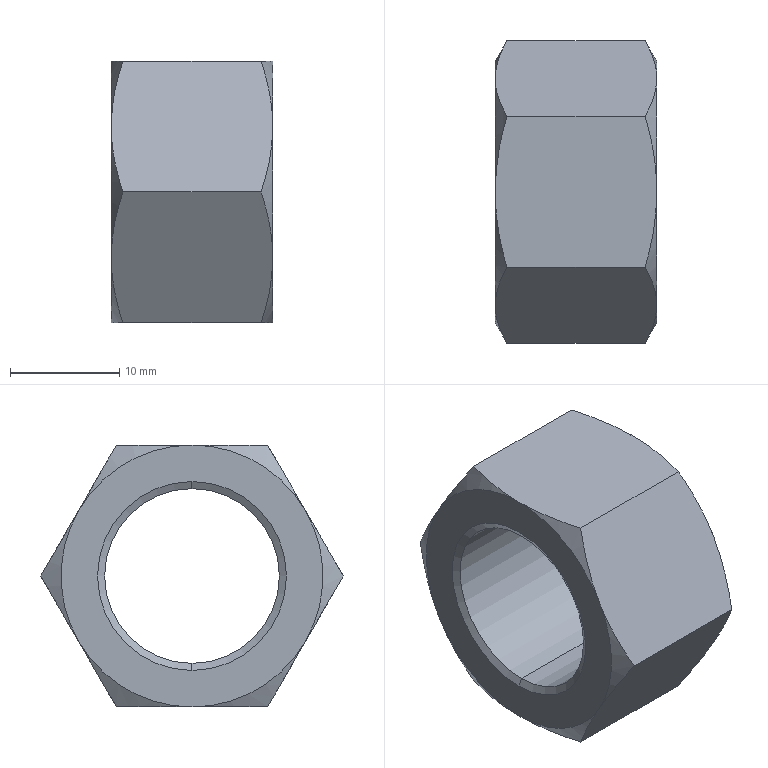Component | SolidWorks | GB_T6170-2015[Type1HexNutM16]-1 | 1 solid | 26 faces | box 14.8 x 27.71 x 24 mm | volume 4364 mm3 | cone 16 | plane 8 | cylinder 2 | commonest cylinder face diameters 16 x2
build123d program:
from build123d import *

# Parameters (mm, degrees)
SKETCH3_R               = 6.918
BOSS_EXTRUDE1_DEPTH     = 14.8
SKETCH5_R               = 20.062
SKETCH5_R_2             = 12
CUT_EXTRUDE1_2_DEPTH    = 2.96
CUT_EXTRUDE1_2_DRAFT    = -60
SKETCH7_R               = 20.062
SKETCH7_R_2             = 12
CUT_EXTRUDE2_DEPTH      = 2.96
CUT_EXTRUDE2_DRAFT      = -60
CUT_EXTRUDE1_DEPTH      = 24.559
CUT_EXTRUDE1_DEPTH_BACK = 24.559
SKETCH1_R               = 8


with BuildPart() as part:
    # Sketch3 → Boss-Extrude1 (new body)
    with BuildSketch(Plane.XY):
        Polygon((0, 13.856), (-12, 6.928), (-12, -6.928), (0, -13.856), (12, -6.928), (12, 6.928), align=None)
        Circle(SKETCH3_R, mode=Mode.SUBTRACT)
    extrude(amount=-BOSS_EXTRUDE1_DEPTH)

    # Sketch4 → Cut-Revolve1 (revolve, cut)
    with BuildSketch(Plane(origin=(0, 0, 0), x_dir=(0, 0, -1), z_dir=(1, 0, 0)), mode=Mode.PRIVATE) as cut_revolve1_sk:
        Polygon((0, 8.65), (1, 6.918), (1, 0), (0, 0), align=None)
        Polygon((14.8, 0), (14.8, 8.65), (13.8, 6.918), (13.8, 0), align=None)
    revolve(cut_revolve1_sk.sketch.rotate(Axis((0, 0, 0), (0, 0, -1)), 90), axis=Axis((0, 0, 0), (0, 0, -1)), mode=Mode.SUBTRACT)


with BuildPart() as cut_extrude1_2_tool:
    # Sketch5 → Cut-Extrude1_2 (with draft: the straight prism first)
    with BuildSketch(Plane.XY):
        Circle(SKETCH5_R)
        Circle(SKETCH5_R_2, mode=Mode.SUBTRACT)
    extrude(amount=-CUT_EXTRUDE1_2_DEPTH)
    # Cut-Extrude1_2: the draft: its side faces are tilted about the plane it starts from
    cut_extrude1_2_sides = [cut_extrude1_2_tool.faces().sort_by_distance(p)[0] for p in [
        (-20.062, 0, -1.48),
        (-12, 0, -1.48),
    ]]
    draft(cut_extrude1_2_sides, Plane.XY, CUT_EXTRUDE1_2_DRAFT)


with BuildPart() as part_1:
    add(part.part)

    # Cut-Extrude1_2: cut by cut_extrude1_2_tool
    add(cut_extrude1_2_tool.part, mode=Mode.SUBTRACT)


with BuildPart() as cut_extrude2_tool:
    # Sketch7 → Cut-Extrude2 (with draft: the straight prism first)
    with BuildSketch(Plane(origin=(0, 0, -14.8), x_dir=(-1, 0, 0), z_dir=(0, 0, -1))):
        Circle(SKETCH7_R)
        Circle(SKETCH7_R_2, mode=Mode.SUBTRACT)
    extrude(amount=-CUT_EXTRUDE2_DEPTH)
    # Cut-Extrude2: the draft: its side faces are tilted about the plane it starts from
    cut_extrude2_sides = [cut_extrude2_tool.faces().sort_by_distance(p)[0] for p in [
        (20.062, 0, -13.32),
        (12, 0, -13.32),
    ]]
    draft(cut_extrude2_sides, Plane(origin=(0, 0, -14.8), x_dir=(-1, 0, 0), z_dir=(0, 0, -1)), CUT_EXTRUDE2_DRAFT)


with BuildPart() as part_2:
    add(part_1.part)

    # Cut-Extrude2: cut by cut_extrude2_tool
    add(cut_extrude2_tool.part, mode=Mode.SUBTRACT)

    # Sketch1 → Cut-Extrude1 (cut, two sides: drawn at the far end of the back side and taken through both)
    with BuildSketch(Plane.XY.offset(-CUT_EXTRUDE1_DEPTH_BACK)):
        Circle(SKETCH1_R)
    extrude(amount=CUT_EXTRUDE1_DEPTH + CUT_EXTRUDE1_DEPTH_BACK, mode=Mode.SUBTRACT)


solid = part_2.part

# Placed as in the assembly
solid = solid.moved(Location((-236.5, 7106.066, 106.066), (0, 90, 0)))
STEP:
#1=COLOUR_RGB('',0.7922,0.8196,0.9333);
#2=FILL_AREA_STYLE_COLOUR('',#1);
#3=FILL_AREA_STYLE('',(#2));
#4=SURFACE_STYLE_FILL_AREA(#3);
#5=SURFACE_SIDE_STYLE('',(#4));
#6=SURFACE_STYLE_USAGE(.BOTH.,#5);
#7=PRESENTATION_STYLE_ASSIGNMENT((#6));
#8=CARTESIAN_POINT('',(-9.326,279.766,4.491));
#9=VERTEX_POINT('',#8);
#10=CARTESIAN_POINT('',(-9.326,279.766,3.861));
#11=VERTEX_POINT('',#10);
#12=CARTESIAN_POINT('',(-9.326,279.766,4.176));
#13=DIRECTION('',(1.,0.,0.));
#14=DIRECTION('',(0.,0.,-1.));
#15=AXIS2_PLACEMENT_3D('',#12,#13,#14);
#16=CIRCLE('',#15,0.315);
#17=EDGE_CURVE('',#9,#11,#16,.T.);
#18=ORIENTED_EDGE('',*,*,#17,.T.);
#19=CARTESIAN_POINT('',(-9.879,279.766,3.861));
#20=VERTEX_POINT('',#19);
#21=CARTESIAN_POINT('',(-9.311,279.766,3.861));
#22=DIRECTION('',(-1.,0.,0.));
#23=VECTOR('',#22,39.37);
#24=LINE('',#21,#23);
#25=EDGE_CURVE('',#11,#20,#24,.T.);
#26=ORIENTED_EDGE('',*,*,#25,.T.);
#27=CARTESIAN_POINT('',(-9.879,279.766,4.491));
#28=VERTEX_POINT('',#27);
#29=CARTESIAN_POINT('',(-9.879,279.766,4.176));
#30=DIRECTION('',(-1.,0.,0.));
#31=DIRECTION('',(0.,0.,1.));
#32=AXIS2_PLACEMENT_3D('',#29,#30,#31);
#33=CIRCLE('',#32,0.315);
#34=EDGE_CURVE('',#20,#28,#33,.T.);
#35=ORIENTED_EDGE('',*,*,#34,.T.);
#36=CARTESIAN_POINT('',(-9.311,279.766,4.491));
#37=DIRECTION('',(-1.,0.,0.));
#38=VECTOR('',#37,39.37);
#39=LINE('',#36,#38);
#40=EDGE_CURVE('',#9,#28,#39,.T.);
#41=ORIENTED_EDGE('',*,*,#40,.F.);
#42=EDGE_LOOP('',(#18,#26,#35,#41));
#43=FACE_OUTER_BOUND('',#42,.T.);
#44=CARTESIAN_POINT('',(-9.311,279.766,4.176));
#45=DIRECTION('',(-1.,0.,0.));
#46=DIRECTION('',(0.,0.,1.));
#47=AXIS2_PLACEMENT_3D('',#44,#45,#46);
#48=CYLINDRICAL_SURFACE('',#47,0.315);
#49=ADVANCED_FACE('',(#43),#48,.F.);
#50=ORIENTED_EDGE('',*,*,#17,.F.);
#51=CARTESIAN_POINT('',(-9.311,279.766,4.516));
#52=VERTEX_POINT('',#51);
#53=CARTESIAN_POINT('',(-9.311,279.766,4.516));
#54=DIRECTION('',(0.5,0.,0.866));
#55=VECTOR('',#54,39.37);
#56=LINE('',#53,#55);
#57=EDGE_CURVE('',#9,#52,#56,.T.);
#58=ORIENTED_EDGE('',*,*,#57,.T.);
#59=CARTESIAN_POINT('',(-9.311,279.766,3.835));
#60=VERTEX_POINT('',#59);
#61=CARTESIAN_POINT('',(-9.311,279.766,4.176));
#62=DIRECTION('',(-1.,0.,0.));
#63=DIRECTION('',(0.,0.,1.));
#64=AXIS2_PLACEMENT_3D('',#61,#62,#63);
#65=CIRCLE('',#64,0.3406);
#66=EDGE_CURVE('',#60,#52,#65,.T.);
#67=ORIENTED_EDGE('',*,*,#66,.F.);
#68=CARTESIAN_POINT('',(-9.311,279.766,3.835));
#69=DIRECTION('',(0.5,0.,-0.866));
#70=VECTOR('',#69,39.37);
#71=LINE('',#68,#70);
#72=EDGE_CURVE('',#11,#60,#71,.T.);
#73=ORIENTED_EDGE('',*,*,#72,.F.);
#74=EDGE_LOOP('',(#50,#58,#67,#73));
#75=FACE_OUTER_BOUND('',#74,.T.);
#76=CARTESIAN_POINT('',(-9.311,279.766,4.176));
#77=DIRECTION('',(1.,0.,0.));
#78=DIRECTION('',(0.,0.,-1.));
#79=AXIS2_PLACEMENT_3D('',#76,#77,#78);
#80=CONICAL_SURFACE('',#79,0.3406,1.047);
#81=ADVANCED_FACE('',(#75),#80,.F.);
#82=ORIENTED_EDGE('',*,*,#34,.F.);
#83=CARTESIAN_POINT('',(-9.894,279.766,3.835));
#84=VERTEX_POINT('',#83);
#85=CARTESIAN_POINT('',(-9.854,279.766,3.903));
#86=DIRECTION('',(-0.5,0.,-0.866));
#87=VECTOR('',#86,39.37);
#88=LINE('',#85,#87);
#89=EDGE_CURVE('',#20,#84,#88,.T.);
#90=ORIENTED_EDGE('',*,*,#89,.T.);
#91=CARTESIAN_POINT('',(-9.894,279.766,4.516));
#92=VERTEX_POINT('',#91);
#93=CARTESIAN_POINT('',(-9.894,279.766,4.176));
#94=DIRECTION('',(-1.,0.,0.));
#95=DIRECTION('',(0.,0.,1.));
#96=AXIS2_PLACEMENT_3D('',#93,#94,#95);
#97=CIRCLE('',#96,0.3406);
#98=EDGE_CURVE('',#84,#92,#97,.T.);
#99=ORIENTED_EDGE('',*,*,#98,.T.);
#100=CARTESIAN_POINT('',(-9.854,279.766,4.448));
#101=DIRECTION('',(-0.5,0.,0.866));
#102=VECTOR('',#101,39.37);
#103=LINE('',#100,#102);
#104=EDGE_CURVE('',#28,#92,#103,.T.);
#105=ORIENTED_EDGE('',*,*,#104,.F.);
#106=EDGE_LOOP('',(#82,#90,#99,#105));
#107=FACE_OUTER_BOUND('',#106,.T.);
#108=CARTESIAN_POINT('',(-9.854,279.766,4.176));
#109=DIRECTION('',(-1.,0.,0.));
#110=DIRECTION('',(0.,0.,1.));
#111=AXIS2_PLACEMENT_3D('',#108,#109,#110);
#112=CONICAL_SURFACE('',#111,0.2723,1.047);
#113=ADVANCED_FACE('',(#107),#112,.F.);
#114=CARTESIAN_POINT('',(-9.353,280.039,4.648));
#115=VERTEX_POINT('',#114);
#116=CARTESIAN_POINT('',(-9.852,280.039,4.648));
#117=VERTEX_POINT('',#116);
#118=CARTESIAN_POINT('',(-9.311,280.039,4.648));
#119=DIRECTION('',(-1.,0.,0.));
#120=VECTOR('',#119,39.37);
#121=LINE('',#118,#120);
#122=EDGE_CURVE('',#115,#117,#121,.T.);
#123=ORIENTED_EDGE('',*,*,#122,.F.);
#124=CARTESIAN_POINT('',(-9.311,280.176,4.412));
#125=VERTEX_POINT('',#124);
#126=CARTESIAN_POINT('',(-9.353,280.039,4.648));
#127=CARTESIAN_POINT('',(-9.34,280.061,4.61));
#128=CARTESIAN_POINT('',(-9.33,280.084,4.571));
#129=CARTESIAN_POINT('',(-9.315,280.129,4.492));
#130=CARTESIAN_POINT('',(-9.311,280.152,4.452));
#131=CARTESIAN_POINT('',(-9.311,280.176,4.412));
#132=B_SPLINE_CURVE_WITH_KNOTS('',3,(#126,#127,#128,#129,#130,#131),.UNSPECIFIED.,.F.,.F.,(4,2,4),(0.00000024,0.003505,0.00701),.UNSPECIFIED.);
#133=EDGE_CURVE('',#115,#125,#132,.T.);
#134=ORIENTED_EDGE('',*,*,#133,.T.);
#135=CARTESIAN_POINT('',(-9.353,280.312,4.176));
#136=VERTEX_POINT('',#135);
#137=CARTESIAN_POINT('',(-9.311,280.176,4.412));
#138=CARTESIAN_POINT('',(-9.311,280.187,4.392));
#139=CARTESIAN_POINT('',(-9.312,280.199,4.372));
#140=CARTESIAN_POINT('',(-9.316,280.222,4.332));
#141=CARTESIAN_POINT('',(-9.319,280.233,4.312));
#142=CARTESIAN_POINT('',(-9.33,280.267,4.253));
#143=CARTESIAN_POINT('',(-9.34,280.29,4.214));
#144=CARTESIAN_POINT('',(-9.353,280.312,4.176));
#145=B_SPLINE_CURVE_WITH_KNOTS('',3,(#137,#138,#139,#140,#141,#142,#143,#144),.UNSPECIFIED.,.F.,.F.,(4,2,2,4),(0.00701,0.008756,0.0105,0.01399),.UNSPECIFIED.);
#146=EDGE_CURVE('',#125,#136,#145,.T.);
#147=ORIENTED_EDGE('',*,*,#146,.T.);
#148=CARTESIAN_POINT('',(-9.852,280.312,4.176));
#149=VERTEX_POINT('',#148);
#150=CARTESIAN_POINT('',(-9.311,280.312,4.176));
#151=DIRECTION('',(-1.,0.,0.));
#152=VECTOR('',#151,39.37);
#153=LINE('',#150,#152);
#154=EDGE_CURVE('',#136,#149,#153,.T.);
#155=ORIENTED_EDGE('',*,*,#154,.T.);
#156=CARTESIAN_POINT('',(-9.894,280.176,4.412));
#157=VERTEX_POINT('',#156);
#158=CARTESIAN_POINT('',(-9.852,280.312,4.176));
#159=CARTESIAN_POINT('',(-9.864,280.29,4.214));
#160=CARTESIAN_POINT('',(-9.875,280.267,4.253));
#161=CARTESIAN_POINT('',(-9.89,280.222,4.332));
#162=CARTESIAN_POINT('',(-9.894,280.199,4.372));
#163=CARTESIAN_POINT('',(-9.894,280.176,4.412));
#164=B_SPLINE_CURVE_WITH_KNOTS('',3,(#158,#159,#160,#161,#162,#163),.UNSPECIFIED.,.F.,.F.,(4,2,4),(0.00000024,0.003505,0.00701),.UNSPECIFIED.);
#165=EDGE_CURVE('',#149,#157,#164,.T.);
#166=ORIENTED_EDGE('',*,*,#165,.T.);
#167=CARTESIAN_POINT('',(-9.894,280.176,4.412));
#168=CARTESIAN_POINT('',(-9.894,280.164,4.432));
#169=CARTESIAN_POINT('',(-9.893,280.152,4.452));
#170=CARTESIAN_POINT('',(-9.889,280.129,4.492));
#171=CARTESIAN_POINT('',(-9.886,280.118,4.512));
#172=CARTESIAN_POINT('',(-9.875,280.084,4.571));
#173=CARTESIAN_POINT('',(-9.864,280.061,4.61));
#174=CARTESIAN_POINT('',(-9.852,280.039,4.648));
#175=B_SPLINE_CURVE_WITH_KNOTS('',3,(#167,#168,#169,#170,#171,#172,#173,#174),.UNSPECIFIED.,.F.,.F.,(4,2,2,4),(0.00701,0.008756,0.0105,0.01399),.UNSPECIFIED.);
#176=EDGE_CURVE('',#157,#117,#175,.T.);
#177=ORIENTED_EDGE('',*,*,#176,.T.);
#178=EDGE_LOOP('',(#123,#134,#147,#155,#166,#177));
#179=FACE_OUTER_BOUND('',#178,.T.);
#180=CARTESIAN_POINT('',(-9.311,280.039,4.648));
#181=DIRECTION('',(0.,0.866,0.5));
#182=DIRECTION('',(0.,0.5,-0.866));
#183=AXIS2_PLACEMENT_3D('',#180,#181,#182);
#184=PLANE('',#183);
#185=ADVANCED_FACE('',(#179),#184,.T.);
#186=CARTESIAN_POINT('',(-9.353,279.494,4.648));
#187=VERTEX_POINT('',#186);
#188=CARTESIAN_POINT('',(-9.852,279.494,4.648));
#189=VERTEX_POINT('',#188);
#190=CARTESIAN_POINT('',(-9.311,279.494,4.648));
#191=DIRECTION('',(-1.,0.,0.));
#192=VECTOR('',#191,39.37);
#193=LINE('',#190,#192);
#194=EDGE_CURVE('',#187,#189,#193,.T.);
#195=ORIENTED_EDGE('',*,*,#194,.F.);
#196=CARTESIAN_POINT('',(-9.311,279.766,4.648));
#197=VERTEX_POINT('',#196);
#198=CARTESIAN_POINT('',(-9.353,279.494,4.648));
#199=CARTESIAN_POINT('',(-9.34,279.538,4.648));
#200=CARTESIAN_POINT('',(-9.33,279.583,4.648));
#201=CARTESIAN_POINT('',(-9.315,279.674,4.648));
#202=CARTESIAN_POINT('',(-9.311,279.72,4.648));
#203=CARTESIAN_POINT('',(-9.311,279.766,4.648));
#204=B_SPLINE_CURVE_WITH_KNOTS('',3,(#198,#199,#200,#201,#202,#203),.UNSPECIFIED.,.F.,.F.,(4,2,4),(0.01255,0.01606,0.01957),.UNSPECIFIED.);
#205=EDGE_CURVE('',#187,#197,#204,.T.);
#206=ORIENTED_EDGE('',*,*,#205,.T.);
#207=CARTESIAN_POINT('',(-9.311,279.766,4.648));
#208=CARTESIAN_POINT('',(-9.311,279.789,4.648));
#209=CARTESIAN_POINT('',(-9.312,279.813,4.648));
#210=CARTESIAN_POINT('',(-9.316,279.859,4.648));
#211=CARTESIAN_POINT('',(-9.319,279.882,4.648));
#212=CARTESIAN_POINT('',(-9.33,279.95,4.648));
#213=CARTESIAN_POINT('',(-9.34,279.995,4.648));
#214=CARTESIAN_POINT('',(-9.353,280.039,4.648));
#215=B_SPLINE_CURVE_WITH_KNOTS('',3,(#207,#208,#209,#210,#211,#212,#213,#214),.UNSPECIFIED.,.F.,.F.,(4,2,2,4),(0.01957,0.02132,0.02307,0.02658),.UNSPECIFIED.);
#216=EDGE_CURVE('',#197,#115,#215,.T.);
#217=ORIENTED_EDGE('',*,*,#216,.T.);
#218=ORIENTED_EDGE('',*,*,#122,.T.);
#219=CARTESIAN_POINT('',(-9.894,279.766,4.648));
#220=VERTEX_POINT('',#219);
#221=CARTESIAN_POINT('',(-9.852,280.039,4.648));
#222=CARTESIAN_POINT('',(-9.864,279.995,4.648));
#223=CARTESIAN_POINT('',(-9.875,279.95,4.648));
#224=CARTESIAN_POINT('',(-9.886,279.882,4.648));
#225=CARTESIAN_POINT('',(-9.889,279.859,4.648));
#226=CARTESIAN_POINT('',(-9.893,279.813,4.648));
#227=CARTESIAN_POINT('',(-9.894,279.789,4.648));
#228=CARTESIAN_POINT('',(-9.894,279.766,4.648));
#229=B_SPLINE_CURVE_WITH_KNOTS('',3,(#221,#222,#223,#224,#225,#226,#227,#228),.UNSPECIFIED.,.F.,.F.,(4,2,2,4),(0.03088,0.03439,0.03615,0.0379),.UNSPECIFIED.);
#230=EDGE_CURVE('',#117,#220,#229,.T.);
#231=ORIENTED_EDGE('',*,*,#230,.T.);
#232=CARTESIAN_POINT('',(-9.894,279.766,4.648));
#233=CARTESIAN_POINT('',(-9.894,279.72,4.648));
#234=CARTESIAN_POINT('',(-9.89,279.674,4.648));
#235=CARTESIAN_POINT('',(-9.875,279.583,4.648));
#236=CARTESIAN_POINT('',(-9.864,279.538,4.648));
#237=CARTESIAN_POINT('',(-9.852,279.494,4.648));
#238=B_SPLINE_CURVE_WITH_KNOTS('',3,(#232,#233,#234,#235,#236,#237),.UNSPECIFIED.,.F.,.F.,(4,2,4),(0.0379,0.04141,0.04492),.UNSPECIFIED.);
#239=EDGE_CURVE('',#220,#189,#238,.T.);
#240=ORIENTED_EDGE('',*,*,#239,.T.);
#241=EDGE_LOOP('',(#195,#206,#217,#218,#231,#240));
#242=FACE_OUTER_BOUND('',#241,.T.);
#243=CARTESIAN_POINT('',(-9.311,279.494,4.648));
#244=DIRECTION('',(0.,0.,1.));
#245=DIRECTION('',(1.,0.,0.));
#246=AXIS2_PLACEMENT_3D('',#243,#244,#245);
#247=PLANE('',#246);
#248=ADVANCED_FACE('',(#242),#247,.T.);
#249=CARTESIAN_POINT('',(-9.353,279.221,4.176));
#250=VERTEX_POINT('',#249);
#251=CARTESIAN_POINT('',(-9.852,279.221,4.176));
#252=VERTEX_POINT('',#251);
#253=CARTESIAN_POINT('',(-9.311,279.221,4.176));
#254=DIRECTION('',(-1.,0.,0.));
#255=VECTOR('',#254,39.37);
#256=LINE('',#253,#255);
#257=EDGE_CURVE('',#250,#252,#256,.T.);
#258=ORIENTED_EDGE('',*,*,#257,.F.);
#259=CARTESIAN_POINT('',(-9.311,279.357,4.412));
#260=VERTEX_POINT('',#259);
#261=CARTESIAN_POINT('',(-9.353,279.221,4.176));
#262=CARTESIAN_POINT('',(-9.34,279.243,4.214));
#263=CARTESIAN_POINT('',(-9.33,279.266,4.253));
#264=CARTESIAN_POINT('',(-9.315,279.311,4.332));
#265=CARTESIAN_POINT('',(-9.311,279.334,4.372));
#266=CARTESIAN_POINT('',(-9.311,279.357,4.412));
#267=B_SPLINE_CURVE_WITH_KNOTS('',3,(#261,#262,#263,#264,#265,#266),.UNSPECIFIED.,.F.,.F.,(4,2,4),(0.00000024,0.003505,0.00701),.UNSPECIFIED.);
#268=EDGE_CURVE('',#250,#260,#267,.T.);
#269=ORIENTED_EDGE('',*,*,#268,.T.);
#270=CARTESIAN_POINT('',(-9.311,279.357,4.412));
#271=CARTESIAN_POINT('',(-9.311,279.369,4.432));
#272=CARTESIAN_POINT('',(-9.312,279.38,4.452));
#273=CARTESIAN_POINT('',(-9.316,279.403,4.492));
#274=CARTESIAN_POINT('',(-9.319,279.415,4.512));
#275=CARTESIAN_POINT('',(-9.33,279.449,4.571));
#276=CARTESIAN_POINT('',(-9.34,279.471,4.61));
#277=CARTESIAN_POINT('',(-9.353,279.494,4.648));
#278=B_SPLINE_CURVE_WITH_KNOTS('',3,(#270,#271,#272,#273,#274,#275,#276,#277),.UNSPECIFIED.,.F.,.F.,(4,2,2,4),(0.00701,0.008756,0.0105,0.01399),.UNSPECIFIED.);
#279=EDGE_CURVE('',#260,#187,#278,.T.);
#280=ORIENTED_EDGE('',*,*,#279,.T.);
#281=ORIENTED_EDGE('',*,*,#194,.T.);
#282=CARTESIAN_POINT('',(-9.894,279.357,4.412));
#283=VERTEX_POINT('',#282);
#284=CARTESIAN_POINT('',(-9.852,279.494,4.648));
#285=CARTESIAN_POINT('',(-9.864,279.471,4.61));
#286=CARTESIAN_POINT('',(-9.875,279.449,4.571));
#287=CARTESIAN_POINT('',(-9.89,279.403,4.492));
#288=CARTESIAN_POINT('',(-9.894,279.38,4.452));
#289=CARTESIAN_POINT('',(-9.894,279.357,4.412));
#290=B_SPLINE_CURVE_WITH_KNOTS('',3,(#284,#285,#286,#287,#288,#289),.UNSPECIFIED.,.F.,.F.,(4,2,4),(0.00000024,0.003505,0.00701),.UNSPECIFIED.);
#291=EDGE_CURVE('',#189,#283,#290,.T.);
#292=ORIENTED_EDGE('',*,*,#291,.T.);
#293=CARTESIAN_POINT('',(-9.894,279.357,4.412));
#294=CARTESIAN_POINT('',(-9.894,279.346,4.392));
#295=CARTESIAN_POINT('',(-9.893,279.334,4.372));
#296=CARTESIAN_POINT('',(-9.889,279.311,4.332));
#297=CARTESIAN_POINT('',(-9.886,279.3,4.312));
#298=CARTESIAN_POINT('',(-9.875,279.266,4.253));
#299=CARTESIAN_POINT('',(-9.864,279.243,4.214));
#300=CARTESIAN_POINT('',(-9.852,279.221,4.176));
#301=B_SPLINE_CURVE_WITH_KNOTS('',3,(#293,#294,#295,#296,#297,#298,#299,#300),.UNSPECIFIED.,.F.,.F.,(4,2,2,4),(0.00701,0.008756,0.0105,0.01399),.UNSPECIFIED.);
#302=EDGE_CURVE('',#283,#252,#301,.T.);
#303=ORIENTED_EDGE('',*,*,#302,.T.);
#304=EDGE_LOOP('',(#258,#269,#280,#281,#292,#303));
#305=FACE_OUTER_BOUND('',#304,.T.);
#306=CARTESIAN_POINT('',(-9.311,279.221,4.176));
#307=DIRECTION('',(0.,-0.866,0.5));
#308=DIRECTION('',(0.,0.5,0.866));
#309=AXIS2_PLACEMENT_3D('',#306,#307,#308);
#310=PLANE('',#309);
#311=ADVANCED_FACE('',(#305),#310,.T.);
#312=CARTESIAN_POINT('',(-9.353,279.494,3.703));
#313=VERTEX_POINT('',#312);
#314=CARTESIAN_POINT('',(-9.852,279.494,3.703));
#315=VERTEX_POINT('',#314);
#316=CARTESIAN_POINT('',(-9.311,279.494,3.703));
#317=DIRECTION('',(-1.,0.,0.));
#318=VECTOR('',#317,39.37);
#319=LINE('',#316,#318);
#320=EDGE_CURVE('',#313,#315,#319,.T.);
#321=ORIENTED_EDGE('',*,*,#320,.F.);
#322=CARTESIAN_POINT('',(-9.311,279.357,3.94));
#323=VERTEX_POINT('',#322);
#324=CARTESIAN_POINT('',(-9.353,279.494,3.703));
#325=CARTESIAN_POINT('',(-9.34,279.471,3.742));
#326=CARTESIAN_POINT('',(-9.33,279.449,3.781));
#327=CARTESIAN_POINT('',(-9.315,279.403,3.86));
#328=CARTESIAN_POINT('',(-9.311,279.38,3.899));
#329=CARTESIAN_POINT('',(-9.311,279.357,3.94));
#330=B_SPLINE_CURVE_WITH_KNOTS('',3,(#324,#325,#326,#327,#328,#329),.UNSPECIFIED.,.F.,.F.,(4,2,4),(0.00000024,0.003505,0.00701),.UNSPECIFIED.);
#331=EDGE_CURVE('',#313,#323,#330,.T.);
#332=ORIENTED_EDGE('',*,*,#331,.T.);
#333=CARTESIAN_POINT('',(-9.311,279.357,3.94));
#334=CARTESIAN_POINT('',(-9.311,279.346,3.96));
#335=CARTESIAN_POINT('',(-9.312,279.334,3.98));
#336=CARTESIAN_POINT('',(-9.316,279.311,4.02));
#337=CARTESIAN_POINT('',(-9.319,279.3,4.039));
#338=CARTESIAN_POINT('',(-9.33,279.266,4.098));
#339=CARTESIAN_POINT('',(-9.34,279.243,4.137));
#340=CARTESIAN_POINT('',(-9.353,279.221,4.176));
#341=B_SPLINE_CURVE_WITH_KNOTS('',3,(#333,#334,#335,#336,#337,#338,#339,#340),.UNSPECIFIED.,.F.,.F.,(4,2,2,4),(0.00701,0.008756,0.0105,0.01399),.UNSPECIFIED.);
#342=EDGE_CURVE('',#323,#250,#341,.T.);
#343=ORIENTED_EDGE('',*,*,#342,.T.);
#344=ORIENTED_EDGE('',*,*,#257,.T.);
#345=CARTESIAN_POINT('',(-9.894,279.357,3.94));
#346=VERTEX_POINT('',#345);
#347=CARTESIAN_POINT('',(-9.852,279.221,4.176));
#348=CARTESIAN_POINT('',(-9.864,279.243,4.137));
#349=CARTESIAN_POINT('',(-9.875,279.266,4.098));
#350=CARTESIAN_POINT('',(-9.89,279.311,4.02));
#351=CARTESIAN_POINT('',(-9.894,279.334,3.98));
#352=CARTESIAN_POINT('',(-9.894,279.357,3.94));
#353=B_SPLINE_CURVE_WITH_KNOTS('',3,(#347,#348,#349,#350,#351,#352),.UNSPECIFIED.,.F.,.F.,(4,2,4),(0.00000024,0.003505,0.00701),.UNSPECIFIED.);
#354=EDGE_CURVE('',#252,#346,#353,.T.);
#355=ORIENTED_EDGE('',*,*,#354,.T.);
#356=CARTESIAN_POINT('',(-9.894,279.357,3.94));
#357=CARTESIAN_POINT('',(-9.894,279.369,3.92));
#358=CARTESIAN_POINT('',(-9.893,279.38,3.899));
#359=CARTESIAN_POINT('',(-9.889,279.403,3.86));
#360=CARTESIAN_POINT('',(-9.886,279.415,3.84));
#361=CARTESIAN_POINT('',(-9.875,279.449,3.781));
#362=CARTESIAN_POINT('',(-9.864,279.471,3.742));
#363=CARTESIAN_POINT('',(-9.852,279.494,3.703));
#364=B_SPLINE_CURVE_WITH_KNOTS('',3,(#356,#357,#358,#359,#360,#361,#362,#363),.UNSPECIFIED.,.F.,.F.,(4,2,2,4),(0.00701,0.008756,0.0105,0.01399),.UNSPECIFIED.);
#365=EDGE_CURVE('',#346,#315,#364,.T.);
#366=ORIENTED_EDGE('',*,*,#365,.T.);
#367=EDGE_LOOP('',(#321,#332,#343,#344,#355,#366));
#368=FACE_OUTER_BOUND('',#367,.T.);
#369=CARTESIAN_POINT('',(-9.311,279.494,3.703));
#370=DIRECTION('',(0.,-0.866,-0.5));
#371=DIRECTION('',(0.,-0.5,0.866));
#372=AXIS2_PLACEMENT_3D('',#369,#370,#371);
#373=PLANE('',#372);
#374=ADVANCED_FACE('',(#368),#373,.T.);
#375=CARTESIAN_POINT('',(-9.353,280.039,3.703));
#376=VERTEX_POINT('',#375);
#377=CARTESIAN_POINT('',(-9.852,280.039,3.703));
#378=VERTEX_POINT('',#377);
#379=CARTESIAN_POINT('',(-9.311,280.039,3.703));
#380=DIRECTION('',(-1.,0.,0.));
#381=VECTOR('',#380,39.37);
#382=LINE('',#379,#381);
#383=EDGE_CURVE('',#376,#378,#382,.T.);
#384=ORIENTED_EDGE('',*,*,#383,.F.);
#385=CARTESIAN_POINT('',(-9.311,279.766,3.703));
#386=VERTEX_POINT('',#385);
#387=CARTESIAN_POINT('',(-9.353,280.039,3.703));
#388=CARTESIAN_POINT('',(-9.34,279.995,3.703));
#389=CARTESIAN_POINT('',(-9.33,279.95,3.703));
#390=CARTESIAN_POINT('',(-9.319,279.882,3.703));
#391=CARTESIAN_POINT('',(-9.316,279.859,3.703));
#392=CARTESIAN_POINT('',(-9.312,279.813,3.703));
#393=CARTESIAN_POINT('',(-9.311,279.789,3.703));
#394=CARTESIAN_POINT('',(-9.311,279.766,3.703));
#395=B_SPLINE_CURVE_WITH_KNOTS('',3,(#387,#388,#389,#390,#391,#392,#393,#394),.UNSPECIFIED.,.F.,.F.,(4,2,2,4),(0.03088,0.03439,0.03615,0.0379),.UNSPECIFIED.);
#396=EDGE_CURVE('',#376,#386,#395,.T.);
#397=ORIENTED_EDGE('',*,*,#396,.T.);
#398=CARTESIAN_POINT('',(-9.311,279.766,3.703));
#399=CARTESIAN_POINT('',(-9.311,279.72,3.703));
#400=CARTESIAN_POINT('',(-9.315,279.674,3.703));
#401=CARTESIAN_POINT('',(-9.33,279.583,3.703));
#402=CARTESIAN_POINT('',(-9.34,279.538,3.703));
#403=CARTESIAN_POINT('',(-9.353,279.494,3.703));
#404=B_SPLINE_CURVE_WITH_KNOTS('',3,(#398,#399,#400,#401,#402,#403),.UNSPECIFIED.,.F.,.F.,(4,2,4),(0.0379,0.04141,0.04492),.UNSPECIFIED.);
#405=EDGE_CURVE('',#386,#313,#404,.T.);
#406=ORIENTED_EDGE('',*,*,#405,.T.);
#407=ORIENTED_EDGE('',*,*,#320,.T.);
#408=CARTESIAN_POINT('',(-9.894,279.766,3.703));
#409=VERTEX_POINT('',#408);
#410=CARTESIAN_POINT('',(-9.852,279.494,3.703));
#411=CARTESIAN_POINT('',(-9.864,279.538,3.703));
#412=CARTESIAN_POINT('',(-9.875,279.583,3.703));
#413=CARTESIAN_POINT('',(-9.89,279.674,3.703));
#414=CARTESIAN_POINT('',(-9.894,279.72,3.703));
#415=CARTESIAN_POINT('',(-9.894,279.766,3.703));
#416=B_SPLINE_CURVE_WITH_KNOTS('',3,(#410,#411,#412,#413,#414,#415),.UNSPECIFIED.,.F.,.F.,(4,2,4),(0.01255,0.01606,0.01957),.UNSPECIFIED.);
#417=EDGE_CURVE('',#315,#409,#416,.T.);
#418=ORIENTED_EDGE('',*,*,#417,.T.);
#419=CARTESIAN_POINT('',(-9.894,279.766,3.703));
#420=CARTESIAN_POINT('',(-9.894,279.789,3.703));
#421=CARTESIAN_POINT('',(-9.893,279.813,3.703));
#422=CARTESIAN_POINT('',(-9.889,279.859,3.703));
#423=CARTESIAN_POINT('',(-9.886,279.882,3.703));
#424=CARTESIAN_POINT('',(-9.875,279.95,3.703));
#425=CARTESIAN_POINT('',(-9.864,279.995,3.703));
#426=CARTESIAN_POINT('',(-9.852,280.039,3.703));
#427=B_SPLINE_CURVE_WITH_KNOTS('',3,(#419,#420,#421,#422,#423,#424,#425,#426),.UNSPECIFIED.,.F.,.F.,(4,2,2,4),(0.01957,0.02132,0.02307,0.02658),.UNSPECIFIED.);
#428=EDGE_CURVE('',#409,#378,#427,.T.);
#429=ORIENTED_EDGE('',*,*,#428,.T.);
#430=EDGE_LOOP('',(#384,#397,#406,#407,#418,#429));
#431=FACE_OUTER_BOUND('',#430,.T.);
#432=CARTESIAN_POINT('',(-9.311,280.039,3.703));
#433=DIRECTION('',(0.,0.,-1.));
#434=DIRECTION('',(-1.,0.,0.));
#435=AXIS2_PLACEMENT_3D('',#432,#433,#434);
#436=PLANE('',#435);
#437=ADVANCED_FACE('',(#431),#436,.T.);
#438=ORIENTED_EDGE('',*,*,#154,.F.);
#439=CARTESIAN_POINT('',(-9.311,280.176,3.94));
#440=VERTEX_POINT('',#439);
#441=CARTESIAN_POINT('',(-9.353,280.312,4.176));
#442=CARTESIAN_POINT('',(-9.34,280.29,4.137));
#443=CARTESIAN_POINT('',(-9.33,280.267,4.098));
#444=CARTESIAN_POINT('',(-9.315,280.222,4.02));
#445=CARTESIAN_POINT('',(-9.311,280.199,3.98));
#446=CARTESIAN_POINT('',(-9.311,280.176,3.94));
#447=B_SPLINE_CURVE_WITH_KNOTS('',3,(#441,#442,#443,#444,#445,#446),.UNSPECIFIED.,.F.,.F.,(4,2,4),(0.00000024,0.003505,0.00701),.UNSPECIFIED.);
#448=EDGE_CURVE('',#136,#440,#447,.T.);
#449=ORIENTED_EDGE('',*,*,#448,.T.);
#450=CARTESIAN_POINT('',(-9.311,280.176,3.94));
#451=CARTESIAN_POINT('',(-9.311,280.164,3.92));
#452=CARTESIAN_POINT('',(-9.312,280.152,3.899));
#453=CARTESIAN_POINT('',(-9.316,280.129,3.86));
#454=CARTESIAN_POINT('',(-9.319,280.118,3.84));
#455=CARTESIAN_POINT('',(-9.33,280.084,3.781));
#456=CARTESIAN_POINT('',(-9.34,280.061,3.742));
#457=CARTESIAN_POINT('',(-9.353,280.039,3.703));
#458=B_SPLINE_CURVE_WITH_KNOTS('',3,(#450,#451,#452,#453,#454,#455,#456,#457),.UNSPECIFIED.,.F.,.F.,(4,2,2,4),(0.00701,0.008756,0.0105,0.01399),.UNSPECIFIED.);
#459=EDGE_CURVE('',#440,#376,#458,.T.);
#460=ORIENTED_EDGE('',*,*,#459,.T.);
#461=ORIENTED_EDGE('',*,*,#383,.T.);
#462=CARTESIAN_POINT('',(-9.894,280.176,3.94));
#463=VERTEX_POINT('',#462);
#464=CARTESIAN_POINT('',(-9.852,280.039,3.703));
#465=CARTESIAN_POINT('',(-9.864,280.061,3.742));
#466=CARTESIAN_POINT('',(-9.875,280.084,3.781));
#467=CARTESIAN_POINT('',(-9.89,280.129,3.86));
#468=CARTESIAN_POINT('',(-9.894,280.152,3.899));
#469=CARTESIAN_POINT('',(-9.894,280.176,3.94));
#470=B_SPLINE_CURVE_WITH_KNOTS('',3,(#464,#465,#466,#467,#468,#469),.UNSPECIFIED.,.F.,.F.,(4,2,4),(0.00000024,0.003505,0.00701),.UNSPECIFIED.);
#471=EDGE_CURVE('',#378,#463,#470,.T.);
#472=ORIENTED_EDGE('',*,*,#471,.T.);
#473=CARTESIAN_POINT('',(-9.894,280.176,3.94));
#474=CARTESIAN_POINT('',(-9.894,280.187,3.96));
#475=CARTESIAN_POINT('',(-9.893,280.199,3.98));
#476=CARTESIAN_POINT('',(-9.889,280.222,4.02));
#477=CARTESIAN_POINT('',(-9.886,280.233,4.039));
#478=CARTESIAN_POINT('',(-9.875,280.267,4.098));
#479=CARTESIAN_POINT('',(-9.864,280.29,4.137));
#480=CARTESIAN_POINT('',(-9.852,280.312,4.176));
#481=B_SPLINE_CURVE_WITH_KNOTS('',3,(#473,#474,#475,#476,#477,#478,#479,#480),.UNSPECIFIED.,.F.,.F.,(4,2,2,4),(0.00701,0.008756,0.0105,0.01399),.UNSPECIFIED.);
#482=EDGE_CURVE('',#463,#149,#481,.T.);
#483=ORIENTED_EDGE('',*,*,#482,.T.);
#484=EDGE_LOOP('',(#438,#449,#460,#461,#472,#483));
#485=FACE_OUTER_BOUND('',#484,.T.);
#486=CARTESIAN_POINT('',(-9.311,280.312,4.176));
#487=DIRECTION('',(0.,0.866,-0.5));
#488=DIRECTION('',(0.,-0.5,-0.866));
#489=AXIS2_PLACEMENT_3D('',#486,#487,#488);
#490=PLANE('',#489);
#491=ADVANCED_FACE('',(#485),#490,.T.);
#492=ORIENTED_EDGE('',*,*,#66,.T.);
#493=CARTESIAN_POINT('',(-9.311,279.766,4.176));
#494=DIRECTION('',(-1.,0.,0.));
#495=DIRECTION('',(0.,0.,1.));
#496=AXIS2_PLACEMENT_3D('',#493,#494,#495);
#497=CIRCLE('',#496,0.3406);
#498=EDGE_CURVE('',#52,#60,#497,.T.);
#499=ORIENTED_EDGE('',*,*,#498,.T.);
#500=EDGE_LOOP('',(#492,#499));
#501=FACE_BOUND('',#500,.T.);
#502=CARTESIAN_POINT('',(-9.311,279.766,4.176));
#503=DIRECTION('',(-1.,0.,0.));
#504=DIRECTION('',(0.,0.,1.));
#505=AXIS2_PLACEMENT_3D('',#502,#503,#504);
#506=CIRCLE('',#505,0.4724);
#507=EDGE_CURVE('',#197,#125,#506,.T.);
#508=ORIENTED_EDGE('',*,*,#507,.F.);
#509=CARTESIAN_POINT('',(-9.311,279.766,4.176));
#510=DIRECTION('',(-1.,0.,0.));
#511=DIRECTION('',(0.,0.,1.));
#512=AXIS2_PLACEMENT_3D('',#509,#510,#511);
#513=CIRCLE('',#512,0.4724);
#514=EDGE_CURVE('',#260,#197,#513,.T.);
#515=ORIENTED_EDGE('',*,*,#514,.F.);
#516=CARTESIAN_POINT('',(-9.311,279.766,4.176));
#517=DIRECTION('',(-1.,0.,0.));
#518=DIRECTION('',(0.,0.,1.));
#519=AXIS2_PLACEMENT_3D('',#516,#517,#518);
#520=CIRCLE('',#519,0.4724);
#521=EDGE_CURVE('',#323,#260,#520,.T.);
#522=ORIENTED_EDGE('',*,*,#521,.F.);
#523=CARTESIAN_POINT('',(-9.311,279.766,4.176));
#524=DIRECTION('',(-1.,0.,0.));
#525=DIRECTION('',(0.,0.,1.));
#526=AXIS2_PLACEMENT_3D('',#523,#524,#525);
#527=CIRCLE('',#526,0.4724);
#528=EDGE_CURVE('',#386,#323,#527,.T.);
#529=ORIENTED_EDGE('',*,*,#528,.F.);
#530=CARTESIAN_POINT('',(-9.311,279.766,4.176));
#531=DIRECTION('',(1.,0.,0.));
#532=DIRECTION('',(0.,0.,-1.));
#533=AXIS2_PLACEMENT_3D('',#530,#531,#532);
#534=CIRCLE('',#533,0.4724);
#535=EDGE_CURVE('',#386,#440,#534,.T.);
#536=ORIENTED_EDGE('',*,*,#535,.T.);
#537=CARTESIAN_POINT('',(-9.311,279.766,4.176));
#538=DIRECTION('',(-1.,0.,0.));
#539=DIRECTION('',(0.,0.,1.));
#540=AXIS2_PLACEMENT_3D('',#537,#538,#539);
#541=CIRCLE('',#540,0.4724);
#542=EDGE_CURVE('',#125,#440,#541,.T.);
#543=ORIENTED_EDGE('',*,*,#542,.F.);
#544=EDGE_LOOP('',(#508,#515,#522,#529,#536,#543));
#545=FACE_OUTER_BOUND('',#544,.T.);
#546=CARTESIAN_POINT('',(-9.311,280.312,4.176));
#547=DIRECTION('',(-1.,0.,0.));
#548=DIRECTION('',(0.,0.,1.));
#549=AXIS2_PLACEMENT_3D('',#546,#547,#548);
#550=PLANE('',#549);
#551=ADVANCED_FACE('',(#501,#545),#550,.F.);
#552=CARTESIAN_POINT('',(-9.894,279.766,4.176));
#553=DIRECTION('',(-1.,0.,0.));
#554=DIRECTION('',(0.,0.,1.));
#555=AXIS2_PLACEMENT_3D('',#552,#553,#554);
#556=CIRCLE('',#555,0.3406);
#557=EDGE_CURVE('',#92,#84,#556,.T.);
#558=ORIENTED_EDGE('',*,*,#557,.F.);
#559=ORIENTED_EDGE('',*,*,#98,.F.);
#560=EDGE_LOOP('',(#558,#559));
#561=FACE_BOUND('',#560,.T.);
#562=CARTESIAN_POINT('',(-9.894,279.766,4.176));
#563=DIRECTION('',(-1.,0.,0.));
#564=DIRECTION('',(0.,0.,1.));
#565=AXIS2_PLACEMENT_3D('',#562,#563,#564);
#566=CIRCLE('',#565,0.4724);
#567=EDGE_CURVE('',#283,#220,#566,.T.);
#568=ORIENTED_EDGE('',*,*,#567,.T.);
#569=CARTESIAN_POINT('',(-9.894,279.766,4.176));
#570=DIRECTION('',(-1.,0.,0.));
#571=DIRECTION('',(0.,0.,1.));
#572=AXIS2_PLACEMENT_3D('',#569,#570,#571);
#573=CIRCLE('',#572,0.4724);
#574=EDGE_CURVE('',#220,#157,#573,.T.);
#575=ORIENTED_EDGE('',*,*,#574,.T.);
#576=CARTESIAN_POINT('',(-9.894,279.766,4.176));
#577=DIRECTION('',(-1.,0.,0.));
#578=DIRECTION('',(0.,0.,1.));
#579=AXIS2_PLACEMENT_3D('',#576,#577,#578);
#580=CIRCLE('',#579,0.4724);
#581=EDGE_CURVE('',#157,#463,#580,.T.);
#582=ORIENTED_EDGE('',*,*,#581,.T.);
#583=CARTESIAN_POINT('',(-9.894,279.766,4.176));
#584=DIRECTION('',(-1.,0.,0.));
#585=DIRECTION('',(0.,0.,1.));
#586=AXIS2_PLACEMENT_3D('',#583,#584,#585);
#587=CIRCLE('',#586,0.4724);
#588=EDGE_CURVE('',#463,#409,#587,.T.);
#589=ORIENTED_EDGE('',*,*,#588,.T.);
#590=CARTESIAN_POINT('',(-9.894,279.766,4.176));
#591=DIRECTION('',(-1.,0.,0.));
#592=DIRECTION('',(0.,0.,1.));
#593=AXIS2_PLACEMENT_3D('',#590,#591,#592);
#594=CIRCLE('',#593,0.4724);
#595=EDGE_CURVE('',#409,#346,#594,.T.);
#596=ORIENTED_EDGE('',*,*,#595,.T.);
#597=CARTESIAN_POINT('',(-9.894,279.766,4.176));
#598=DIRECTION('',(-1.,0.,0.));
#599=DIRECTION('',(0.,0.,1.));
#600=AXIS2_PLACEMENT_3D('',#597,#598,#599);
#601=CIRCLE('',#600,0.4724);
#602=EDGE_CURVE('',#346,#283,#601,.T.);
#603=ORIENTED_EDGE('',*,*,#602,.T.);
#604=EDGE_LOOP('',(#568,#575,#582,#589,#596,#603));
#605=FACE_OUTER_BOUND('',#604,.T.);
#606=CARTESIAN_POINT('',(-9.894,280.312,4.176));
#607=DIRECTION('',(-1.,0.,0.));
#608=DIRECTION('',(0.,0.,1.));
#609=AXIS2_PLACEMENT_3D('',#606,#607,#608);
#610=PLANE('',#609);
#611=ADVANCED_FACE('',(#561,#605),#610,.T.);
#612=ORIENTED_EDGE('',*,*,#89,.F.);
#613=CARTESIAN_POINT('',(-9.879,279.766,4.176));
#614=DIRECTION('',(-1.,0.,0.));
#615=DIRECTION('',(0.,0.,1.));
#616=AXIS2_PLACEMENT_3D('',#613,#614,#615);
#617=CIRCLE('',#616,0.315);
#618=EDGE_CURVE('',#28,#20,#617,.T.);
#619=ORIENTED_EDGE('',*,*,#618,.F.);
#620=ORIENTED_EDGE('',*,*,#104,.T.);
#621=ORIENTED_EDGE('',*,*,#557,.T.);
#622=EDGE_LOOP('',(#612,#619,#620,#621));
#623=FACE_OUTER_BOUND('',#622,.T.);
#624=CARTESIAN_POINT('',(-9.854,279.766,4.176));
#625=DIRECTION('',(-1.,0.,0.));
#626=DIRECTION('',(0.,0.,1.));
#627=AXIS2_PLACEMENT_3D('',#624,#625,#626);
#628=CONICAL_SURFACE('',#627,0.2723,1.047);
#629=ADVANCED_FACE('',(#623),#628,.F.);
#630=ORIENTED_EDGE('',*,*,#57,.F.);
#631=CARTESIAN_POINT('',(-9.326,279.766,4.176));
#632=DIRECTION('',(1.,0.,0.));
#633=DIRECTION('',(0.,0.,-1.));
#634=AXIS2_PLACEMENT_3D('',#631,#632,#633);
#635=CIRCLE('',#634,0.315);
#636=EDGE_CURVE('',#11,#9,#635,.T.);
#637=ORIENTED_EDGE('',*,*,#636,.F.);
#638=ORIENTED_EDGE('',*,*,#72,.T.);
#639=ORIENTED_EDGE('',*,*,#498,.F.);
#640=EDGE_LOOP('',(#630,#637,#638,#639));
#641=FACE_OUTER_BOUND('',#640,.T.);
#642=CARTESIAN_POINT('',(-9.311,279.766,4.176));
#643=DIRECTION('',(1.,0.,0.));
#644=DIRECTION('',(0.,0.,-1.));
#645=AXIS2_PLACEMENT_3D('',#642,#643,#644);
#646=CONICAL_SURFACE('',#645,0.3406,1.047);
#647=ADVANCED_FACE('',(#641),#646,.F.);
#648=ORIENTED_EDGE('',*,*,#482,.F.);
#649=ORIENTED_EDGE('',*,*,#581,.F.);
#650=ORIENTED_EDGE('',*,*,#165,.F.);
#651=EDGE_LOOP('',(#648,#649,#650));
#652=FACE_OUTER_BOUND('',#651,.T.);
#653=CARTESIAN_POINT('',(-9.894,279.766,4.176));
#654=DIRECTION('',(1.,0.,0.));
#655=DIRECTION('',(0.,0.,1.));
#656=AXIS2_PLACEMENT_3D('',#653,#654,#655);
#657=CONICAL_SURFACE('',#656,0.4724,1.047);
#658=ADVANCED_FACE('',(#652),#657,.T.);
#659=ORIENTED_EDGE('',*,*,#588,.F.);
#660=ORIENTED_EDGE('',*,*,#471,.F.);
#661=ORIENTED_EDGE('',*,*,#428,.F.);
#662=EDGE_LOOP('',(#659,#660,#661));
#663=FACE_OUTER_BOUND('',#662,.T.);
#664=CARTESIAN_POINT('',(-9.894,279.766,4.176));
#665=DIRECTION('',(1.,0.,0.));
#666=DIRECTION('',(0.,0.,1.));
#667=AXIS2_PLACEMENT_3D('',#664,#665,#666);
#668=CONICAL_SURFACE('',#667,0.4724,1.047);
#669=ADVANCED_FACE('',(#663),#668,.T.);
#670=ORIENTED_EDGE('',*,*,#595,.F.);
#671=ORIENTED_EDGE('',*,*,#417,.F.);
#672=ORIENTED_EDGE('',*,*,#365,.F.);
#673=EDGE_LOOP('',(#670,#671,#672));
#674=FACE_OUTER_BOUND('',#673,.T.);
#675=CARTESIAN_POINT('',(-9.894,279.766,4.176));
#676=DIRECTION('',(1.,0.,0.));
#677=DIRECTION('',(0.,0.,1.));
#678=AXIS2_PLACEMENT_3D('',#675,#676,#677);
#679=CONICAL_SURFACE('',#678,0.4724,1.047);
#680=ADVANCED_FACE('',(#674),#679,.T.);
#681=ORIENTED_EDGE('',*,*,#602,.F.);
#682=ORIENTED_EDGE('',*,*,#354,.F.);
#683=ORIENTED_EDGE('',*,*,#302,.F.);
#684=EDGE_LOOP('',(#681,#682,#683));
#685=FACE_OUTER_BOUND('',#684,.T.);
#686=CARTESIAN_POINT('',(-9.894,279.766,4.176));
#687=DIRECTION('',(1.,0.,0.));
#688=DIRECTION('',(0.,0.,1.));
#689=AXIS2_PLACEMENT_3D('',#686,#687,#688);
#690=CONICAL_SURFACE('',#689,0.4724,1.047);
#691=ADVANCED_FACE('',(#685),#690,.T.);
#692=ORIENTED_EDGE('',*,*,#567,.F.);
#693=ORIENTED_EDGE('',*,*,#291,.F.);
#694=ORIENTED_EDGE('',*,*,#239,.F.);
#695=EDGE_LOOP('',(#692,#693,#694));
#696=FACE_OUTER_BOUND('',#695,.T.);
#697=CARTESIAN_POINT('',(-9.894,279.766,4.176));
#698=DIRECTION('',(1.,0.,0.));
#699=DIRECTION('',(0.,0.,1.));
#700=AXIS2_PLACEMENT_3D('',#697,#698,#699);
#701=CONICAL_SURFACE('',#700,0.4724,1.047);
#702=ADVANCED_FACE('',(#696),#701,.T.);
#703=ORIENTED_EDGE('',*,*,#574,.F.);
#704=ORIENTED_EDGE('',*,*,#230,.F.);
#705=ORIENTED_EDGE('',*,*,#176,.F.);
#706=EDGE_LOOP('',(#703,#704,#705));
#707=FACE_OUTER_BOUND('',#706,.T.);
#708=CARTESIAN_POINT('',(-9.894,279.766,4.176));
#709=DIRECTION('',(1.,0.,0.));
#710=DIRECTION('',(0.,0.,1.));
#711=AXIS2_PLACEMENT_3D('',#708,#709,#710);
#712=CONICAL_SURFACE('',#711,0.4724,1.047);
#713=ADVANCED_FACE('',(#707),#712,.T.);
#714=ORIENTED_EDGE('',*,*,#514,.T.);
#715=ORIENTED_EDGE('',*,*,#205,.F.);
#716=ORIENTED_EDGE('',*,*,#279,.F.);
#717=EDGE_LOOP('',(#714,#715,#716));
#718=FACE_OUTER_BOUND('',#717,.T.);
#719=CARTESIAN_POINT('',(-9.311,279.766,4.176));
#720=DIRECTION('',(-1.,0.,0.));
#721=DIRECTION('',(0.,0.,-1.));
#722=AXIS2_PLACEMENT_3D('',#719,#720,#721);
#723=CONICAL_SURFACE('',#722,0.4724,1.047);
#724=ADVANCED_FACE('',(#718),#723,.T.);
#725=ORIENTED_EDGE('',*,*,#342,.F.);
#726=ORIENTED_EDGE('',*,*,#521,.T.);
#727=ORIENTED_EDGE('',*,*,#268,.F.);
#728=EDGE_LOOP('',(#725,#726,#727));
#729=FACE_OUTER_BOUND('',#728,.T.);
#730=CARTESIAN_POINT('',(-9.311,279.766,4.176));
#731=DIRECTION('',(-1.,0.,0.));
#732=DIRECTION('',(0.,0.,-1.));
#733=AXIS2_PLACEMENT_3D('',#730,#731,#732);
#734=CONICAL_SURFACE('',#733,0.4724,1.047);
#735=ADVANCED_FACE('',(#729),#734,.T.);
#736=ORIENTED_EDGE('',*,*,#405,.F.);
#737=ORIENTED_EDGE('',*,*,#528,.T.);
#738=ORIENTED_EDGE('',*,*,#331,.F.);
#739=EDGE_LOOP('',(#736,#737,#738));
#740=FACE_OUTER_BOUND('',#739,.T.);
#741=CARTESIAN_POINT('',(-9.311,279.766,4.176));
#742=DIRECTION('',(-1.,0.,0.));
#743=DIRECTION('',(0.,0.,-1.));
#744=AXIS2_PLACEMENT_3D('',#741,#742,#743);
#745=CONICAL_SURFACE('',#744,0.4724,1.047);
#746=ADVANCED_FACE('',(#740),#745,.T.);
#747=ORIENTED_EDGE('',*,*,#459,.F.);
#748=ORIENTED_EDGE('',*,*,#535,.F.);
#749=ORIENTED_EDGE('',*,*,#396,.F.);
#750=EDGE_LOOP('',(#747,#748,#749));
#751=FACE_OUTER_BOUND('',#750,.T.);
#752=CARTESIAN_POINT('',(-9.311,279.766,4.176));
#753=DIRECTION('',(-1.,0.,0.));
#754=DIRECTION('',(0.,0.,-1.));
#755=AXIS2_PLACEMENT_3D('',#752,#753,#754);
#756=CONICAL_SURFACE('',#755,0.4724,1.047);
#757=ADVANCED_FACE('',(#751),#756,.T.);
#758=ORIENTED_EDGE('',*,*,#542,.T.);
#759=ORIENTED_EDGE('',*,*,#448,.F.);
#760=ORIENTED_EDGE('',*,*,#146,.F.);
#761=EDGE_LOOP('',(#758,#759,#760));
#762=FACE_OUTER_BOUND('',#761,.T.);
#763=CARTESIAN_POINT('',(-9.311,279.766,4.176));
#764=DIRECTION('',(-1.,0.,0.));
#765=DIRECTION('',(0.,0.,-1.));
#766=AXIS2_PLACEMENT_3D('',#763,#764,#765);
#767=CONICAL_SURFACE('',#766,0.4724,1.047);
#768=ADVANCED_FACE('',(#762),#767,.T.);
#769=ORIENTED_EDGE('',*,*,#507,.T.);
#770=ORIENTED_EDGE('',*,*,#133,.F.);
#771=ORIENTED_EDGE('',*,*,#216,.F.);
#772=EDGE_LOOP('',(#769,#770,#771));
#773=FACE_OUTER_BOUND('',#772,.T.);
#774=CARTESIAN_POINT('',(-9.311,279.766,4.176));
#775=DIRECTION('',(-1.,0.,0.));
#776=DIRECTION('',(0.,0.,-1.));
#777=AXIS2_PLACEMENT_3D('',#774,#775,#776);
#778=CONICAL_SURFACE('',#777,0.4724,1.047);
#779=ADVANCED_FACE('',(#773),#778,.T.);
#780=ORIENTED_EDGE('',*,*,#25,.F.);
#781=ORIENTED_EDGE('',*,*,#636,.T.);
#782=ORIENTED_EDGE('',*,*,#40,.T.);
#783=ORIENTED_EDGE('',*,*,#618,.T.);
#784=EDGE_LOOP('',(#780,#781,#782,#783));
#785=FACE_OUTER_BOUND('',#784,.T.);
#786=CARTESIAN_POINT('',(-9.311,279.766,4.176));
#787=DIRECTION('',(-1.,0.,0.));
#788=DIRECTION('',(0.,0.,1.));
#789=AXIS2_PLACEMENT_3D('',#786,#787,#788);
#790=CYLINDRICAL_SURFACE('',#789,0.315);
#791=ADVANCED_FACE('',(#785),#790,.F.);
#792=CLOSED_SHELL('',(#49,#81,#113,#185,#248,#311,#374,#437,#491,#551,#611,#629,#647,#658,#669,#680,#691,#702,#713,#724,#735,#746,#757,#768,#779,#791));
#793=MANIFOLD_SOLID_BREP('',#792);
#794=STYLED_ITEM('',(#7),#793);
#795=(LENGTH_UNIT()NAMED_UNIT(*)SI_UNIT($,.METRE.));
#796=LENGTH_MEASURE_WITH_UNIT(LENGTH_MEASURE(0.0254),#795);
#797=DIMENSIONAL_EXPONENTS(1.,0.,0.,0.,0.,0.,0.);
#798=(CONVERSION_BASED_UNIT('',#796)LENGTH_UNIT()NAMED_UNIT(#797));
#799=UNCERTAINTY_MEASURE_WITH_UNIT(LENGTH_MEASURE(0.00001),#798,'','');
#800=(NAMED_UNIT(*)PLANE_ANGLE_UNIT()SI_UNIT($,.RADIAN.));
#801=(NAMED_UNIT(*)SI_UNIT($,.STERADIAN.)SOLID_ANGLE_UNIT());
#802=(GEOMETRIC_REPRESENTATION_CONTEXT(3)GLOBAL_UNCERTAINTY_ASSIGNED_CONTEXT((#799))GLOBAL_UNIT_ASSIGNED_CONTEXT((#798,#800,#801))REPRESENTATION_CONTEXT('',''));
#803=MECHANICAL_DESIGN_GEOMETRIC_PRESENTATION_REPRESENTATION('',(#794),#802);
#804=CARTESIAN_POINT('',(0.,0.,0.));
#805=DIRECTION('',(0.,0.,1.));
#806=DIRECTION('',(1.,0.,0.));
#807=AXIS2_PLACEMENT_3D('',#804,#805,#806);
#808=(LENGTH_UNIT()NAMED_UNIT(*)SI_UNIT($,.METRE.));
#809=LENGTH_MEASURE_WITH_UNIT(LENGTH_MEASURE(0.0254),#808);
#810=DIMENSIONAL_EXPONENTS(1.,0.,0.,0.,0.,0.,0.);
#811=(CONVERSION_BASED_UNIT('',#809)LENGTH_UNIT()NAMED_UNIT(#810));
#812=UNCERTAINTY_MEASURE_WITH_UNIT(LENGTH_MEASURE(0.00001),#811,'','');
#813=(NAMED_UNIT(*)PLANE_ANGLE_UNIT()SI_UNIT($,.RADIAN.));
#814=(NAMED_UNIT(*)SI_UNIT($,.STERADIAN.)SOLID_ANGLE_UNIT());
#815=(GEOMETRIC_REPRESENTATION_CONTEXT(3)GLOBAL_UNCERTAINTY_ASSIGNED_CONTEXT((#812))GLOBAL_UNIT_ASSIGNED_CONTEXT((#811,#813,#814))REPRESENTATION_CONTEXT('',''));
#816=ADVANCED_BREP_SHAPE_REPRESENTATION('',(#793,#807),#815);
#817=PRESENTATION_LAYER_ASSIGNMENT('','',(#794));